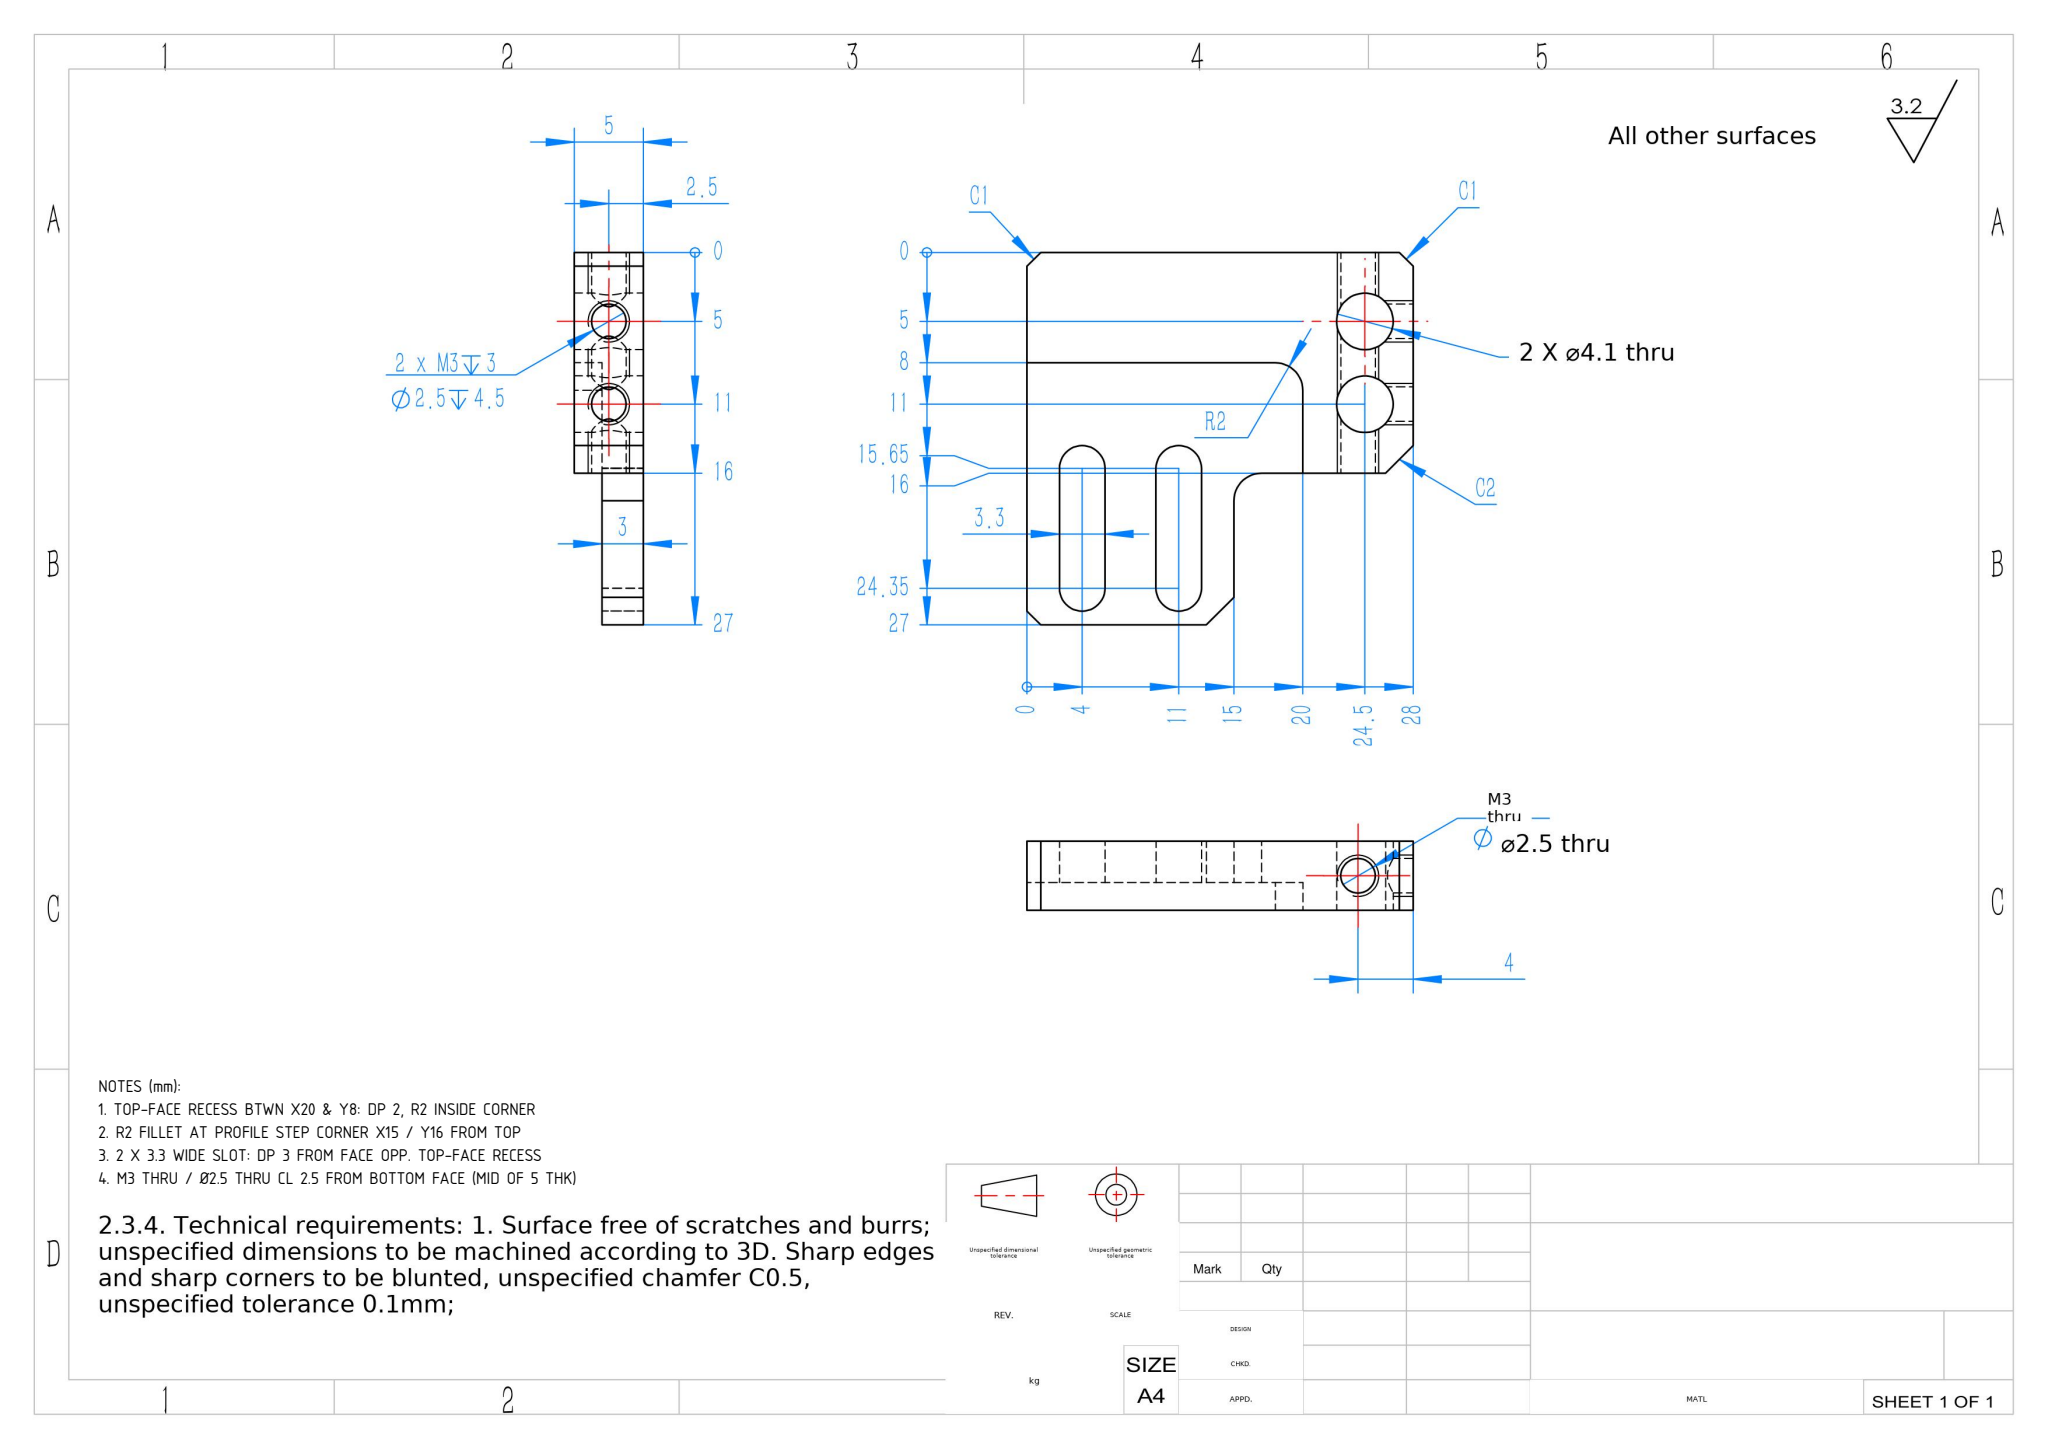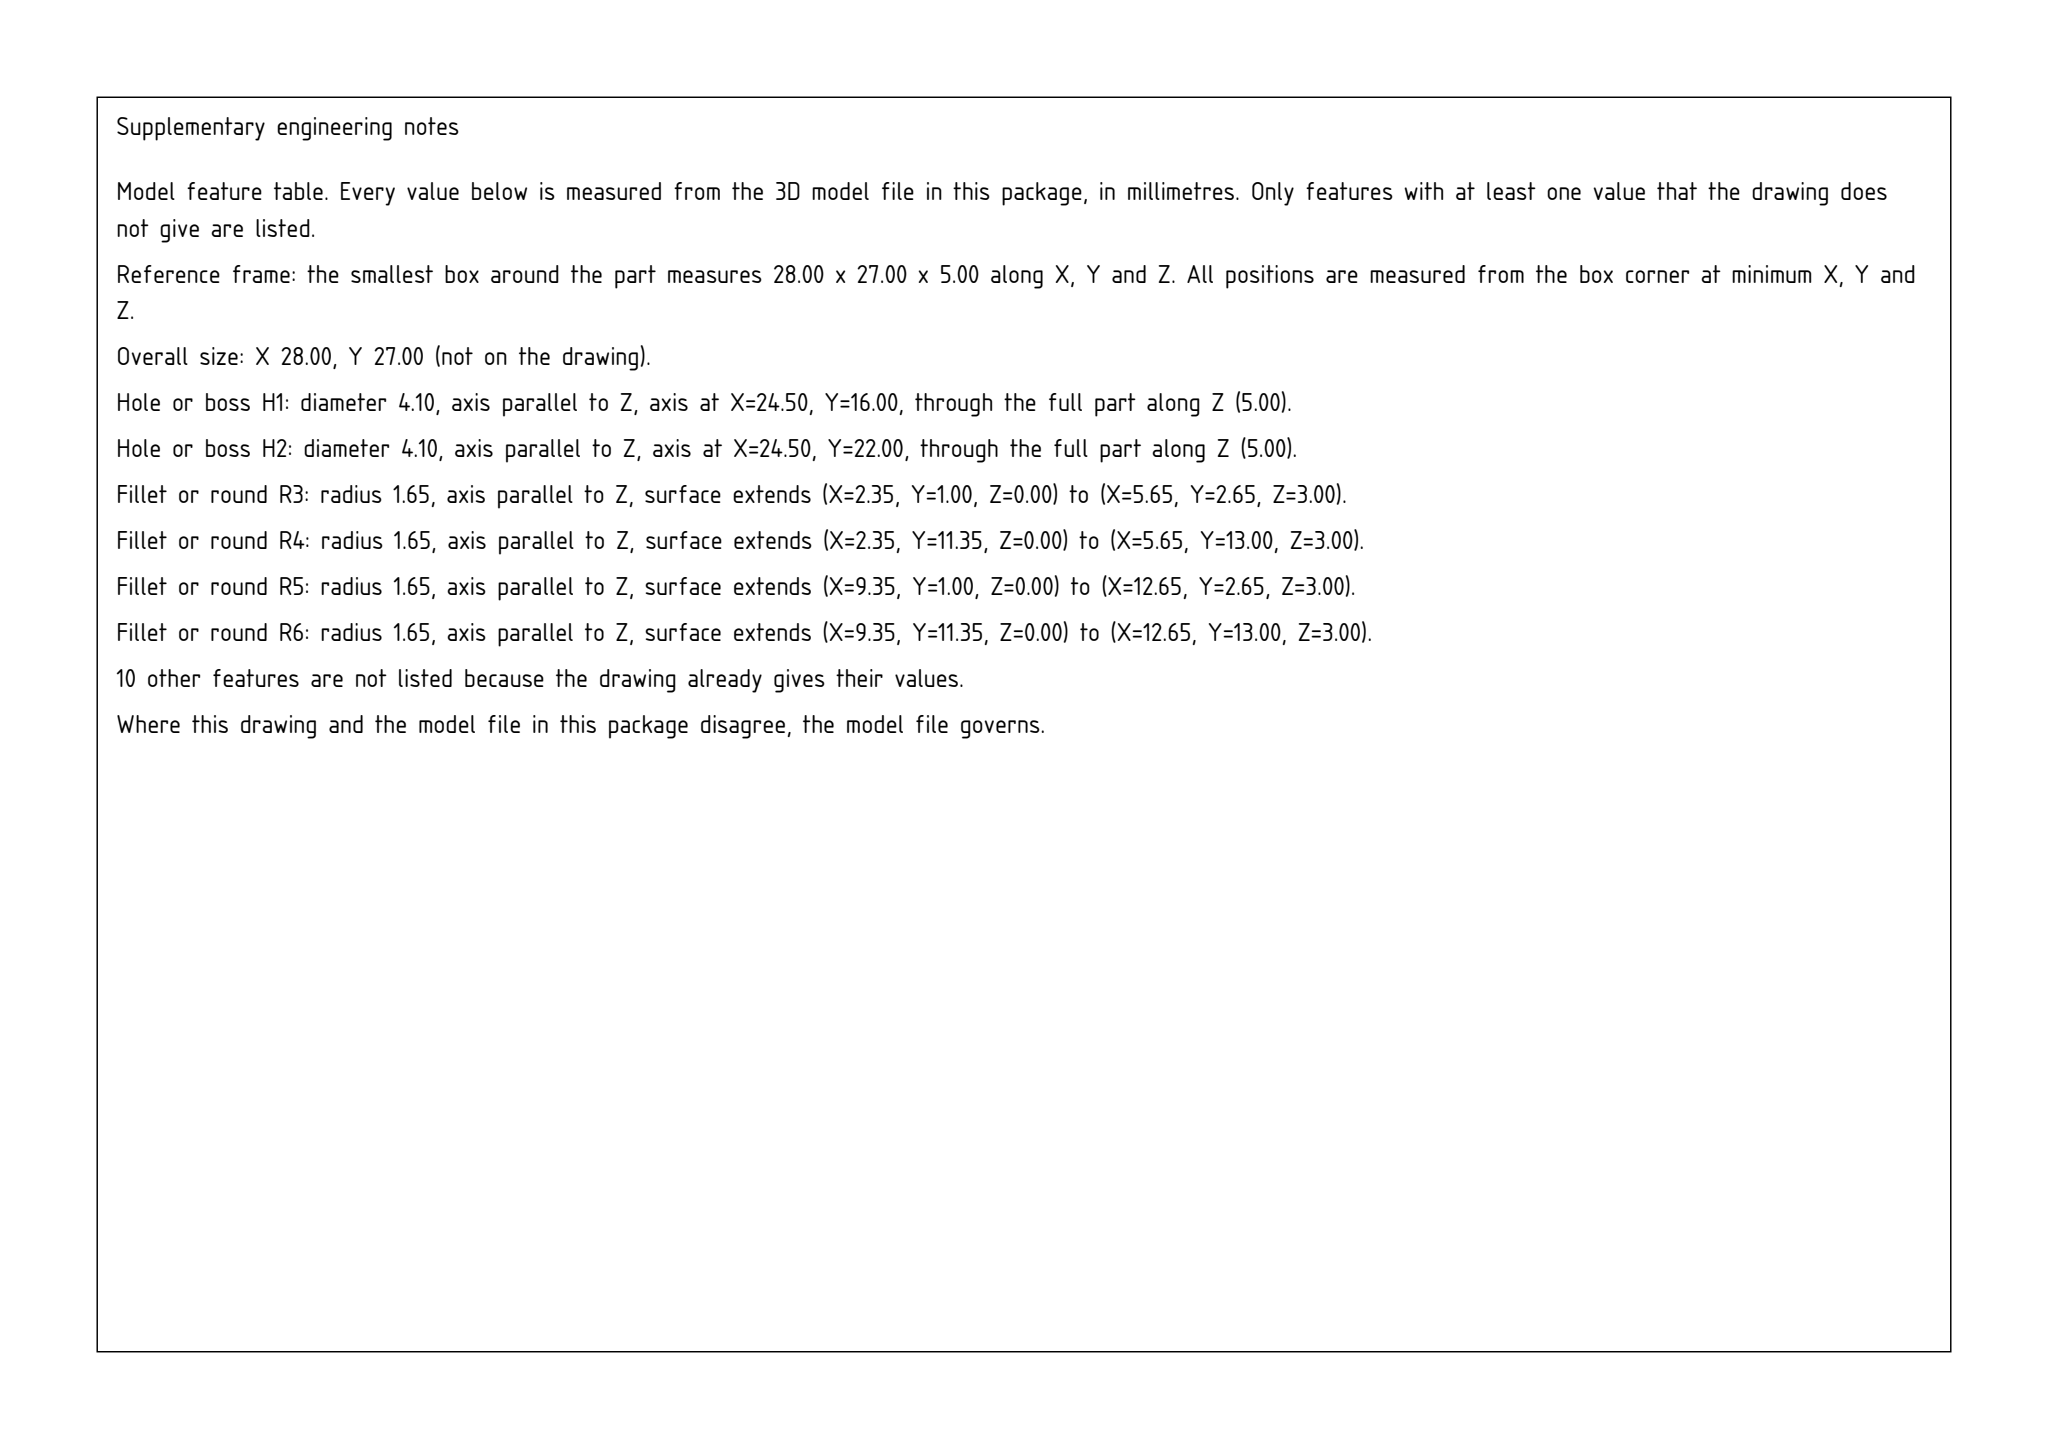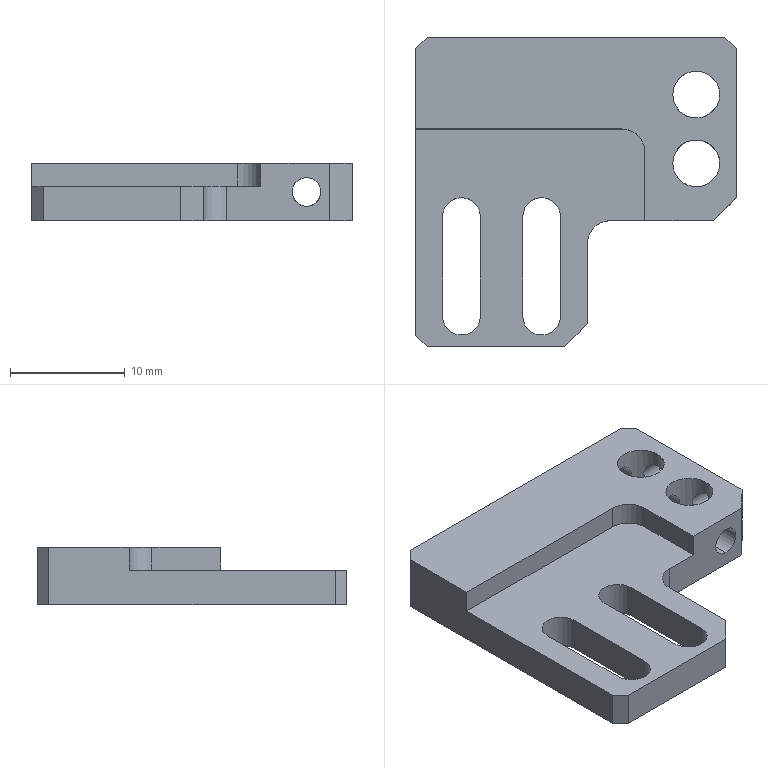Part | SolidWorks | mm | 1 solid | 40 faces | box 28 x 27 x 5 mm | volume 1984 mm3 | cylinder 20 | plane 20 | commonest cylinder face diameters 2.5 x10 4.1 x4 3.3 x4 4 x2
Drawing notes:
TOP-FACE RECESS BTWN X20 & Y8: DP 2, R2 INSIDE CORNER | from the solid: z planes 0/3/5: floor z=3 vs top z=5 = 2 deep; bounded x=20, y=19 (=8 from top); Ø4 z-cyl at (18,17) = R2 corner
R2 FILLET AT PROFILE STEP CORNER X15 / Y16 FROM TOP | from the solid: Planes x=15 and y=11 (=16 from top of bbox Y=27) meet at inside step corner; Ø4 z-cyl at (17,9) = R2
2 X 3.3 WIDE SLOT: DP 3 FROM FACE OPP. TOP-FACE RECESS | from the solid: Ø3.3 z-axis cyls L=3.0 at x=4 & x=11; z planes 0/3/5, recess 2 deep from z=5
M3 THRU / Ø2.5 THRU CL 2.5 FROM BOTTOM FACE (MID OF 5 THK) | from the solid: Ø2.5 y-axis cyls at [x=24.0, z=2.5]; bbox Z = 5.0